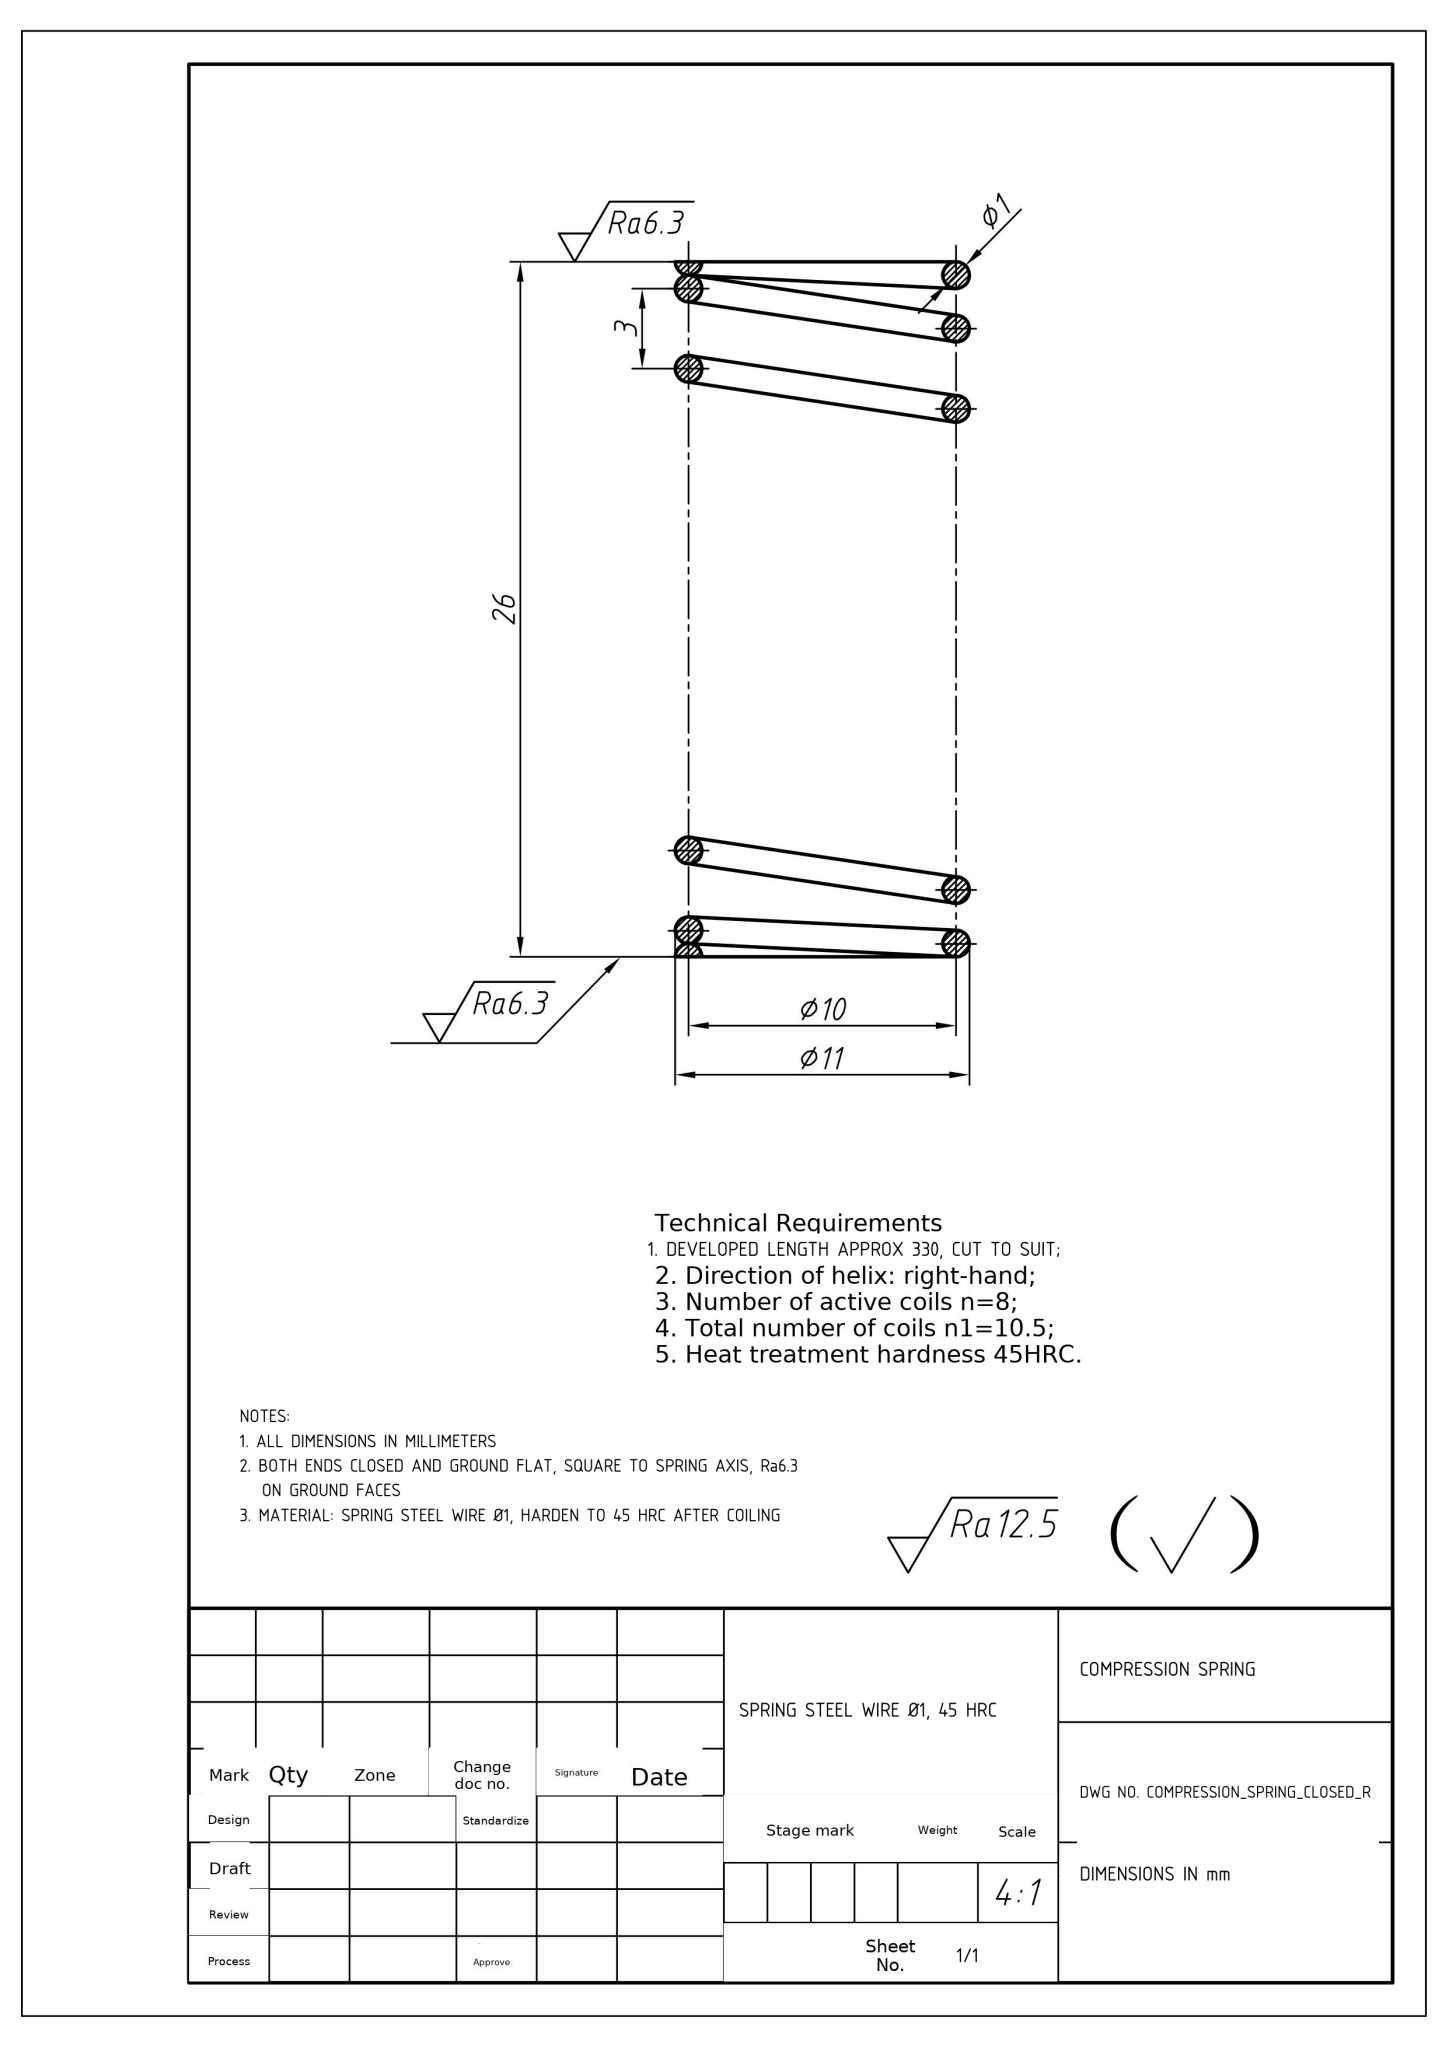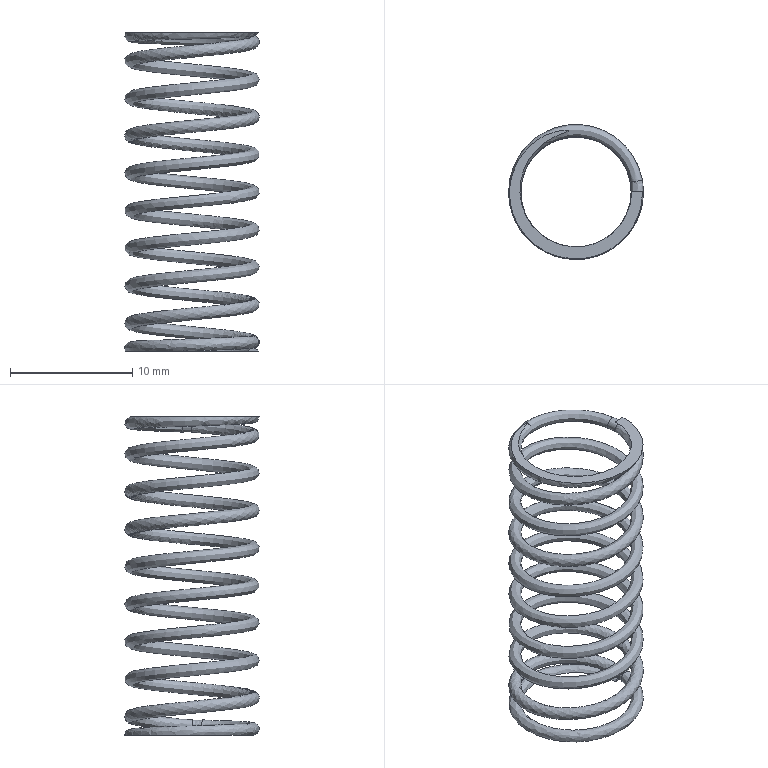Part | NX | mm | 1 solid | 9 faces | box 11 x 10.99 x 27.5 mm | volume 241 mm3 | spline 5 | plane 4